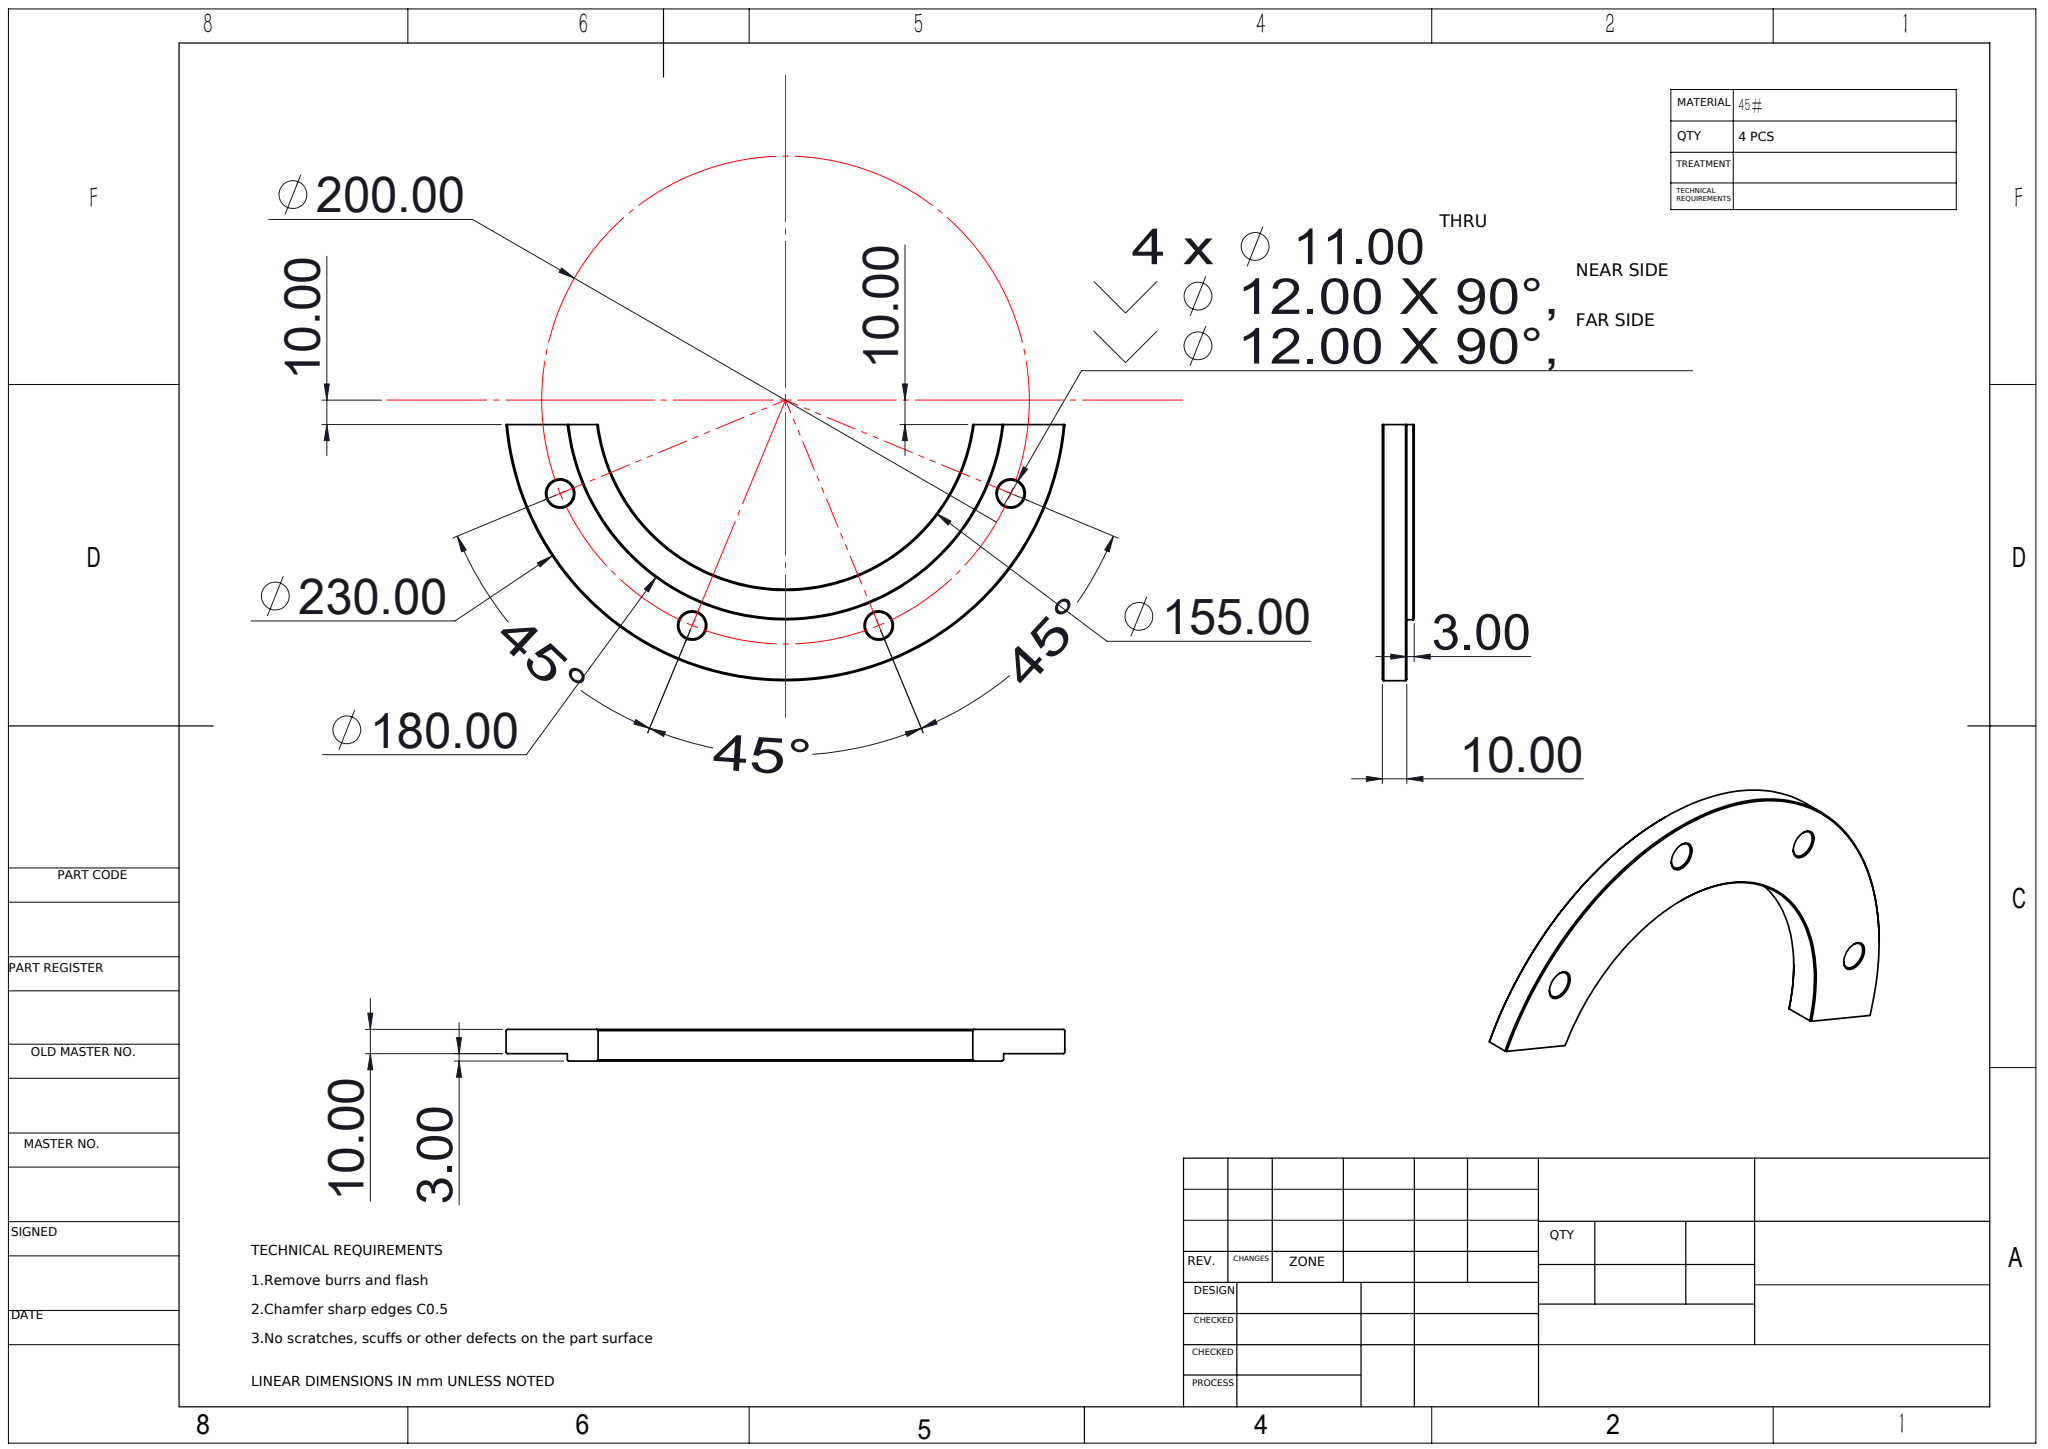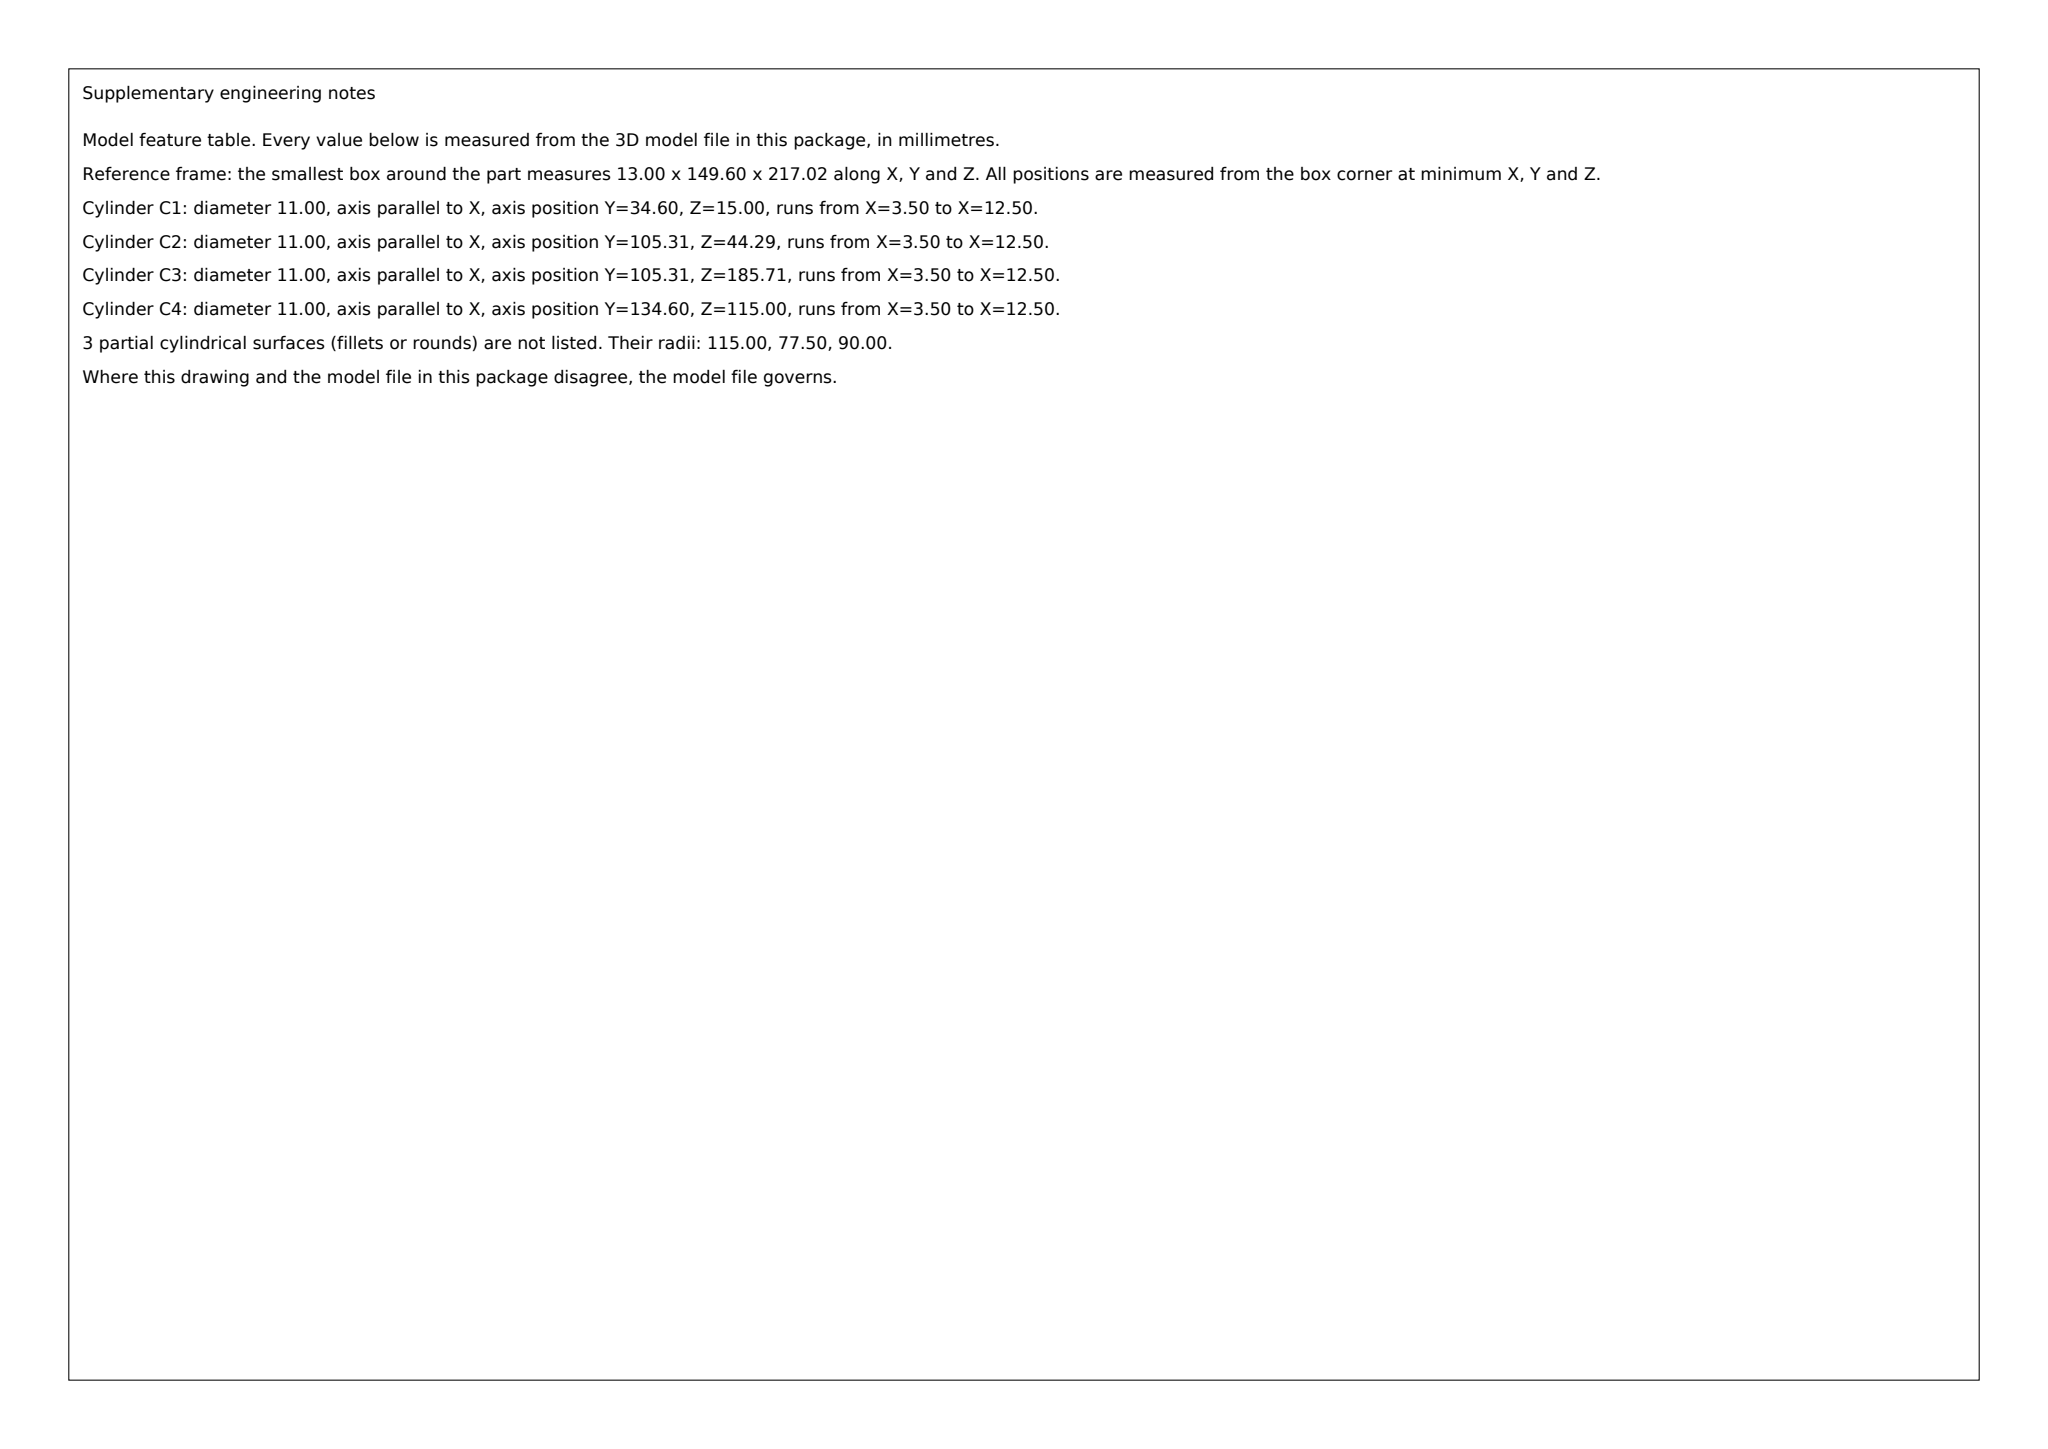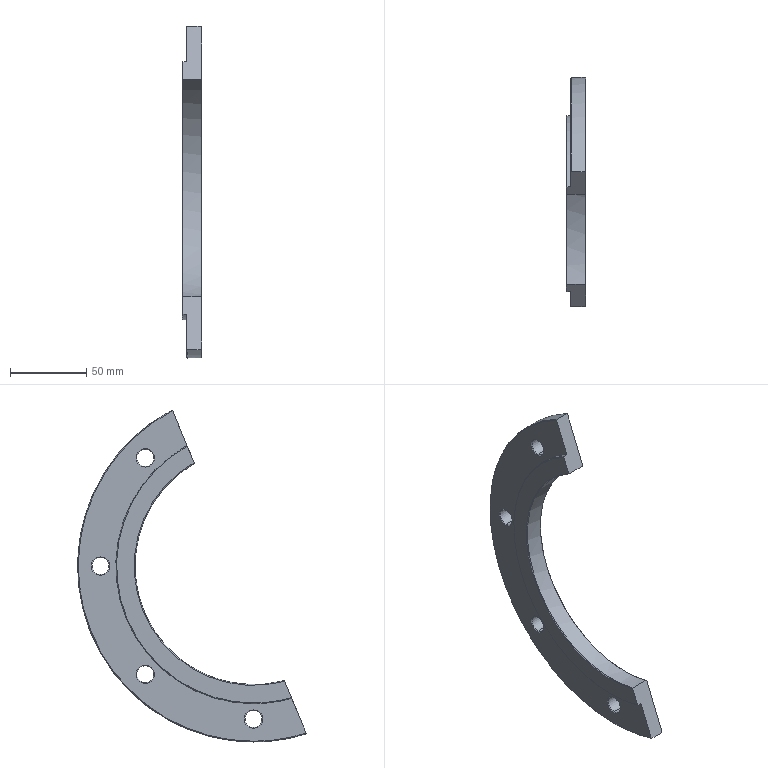Part | SolidWorks | mm | material 45# | 1 solid | 41 faces | box 13 x 149.6 x 217.02 mm | volume 110982 mm3 | cone 24 | cylinder 12 | plane 5 | commonest cylinder face diameters 11 x8 180 x2 230 x1 155 x1